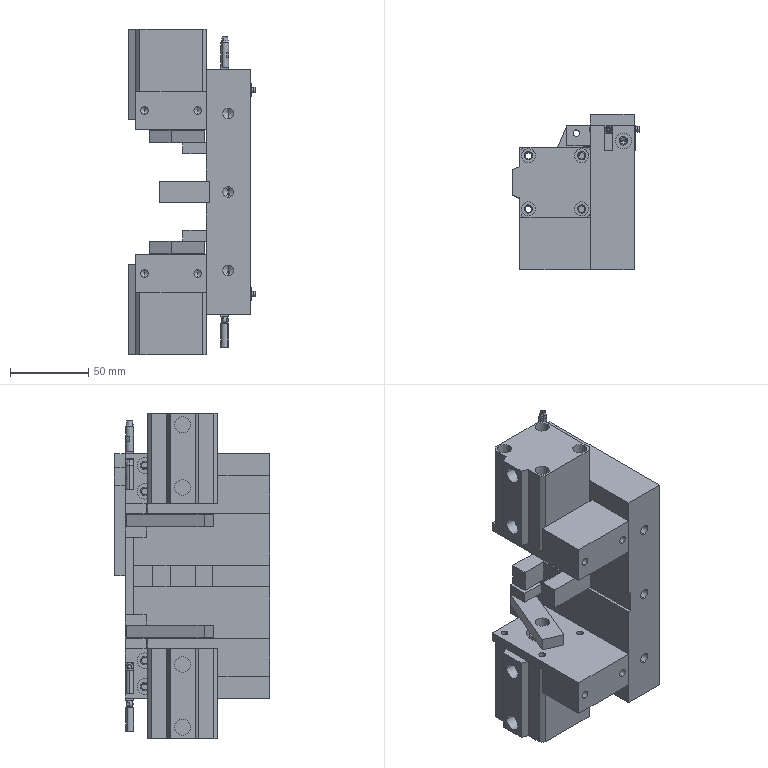Assembly | SolidWorks | mm | 25 component files | 25 solids | 563 faces | box 80.7 x 99 x 208 mm | volume 743615 mm3 | plane 256 | cylinder 242 | cone 53 | sphere 12 | commonest cylinder face diameters 4.2 x44 9 x36 3.5 x24 10 x24 5.5 x20 5.2 x16 4.9 x12 5 x8
Bill of materials:
ACQS-32X25CylinderBody | 2 |  | Square prismatic block with chamfered vertical corners, four corner holes, a larger central bore on the top face, and a trapezoidal tab sticking out from one side.
ACQS-32X25PistonRod | 2 |  | Plain cylindrical tube or sleeve with a concentric bore and flat ends.
InspectionPart | 2 |  | Solid cylindrical pin with a narrow ring-shaped groove of smaller diameter near one end, leaving a short collar at the tip.
PointedHead | 3 |  | Cylindrical shaft with a tapered (conical) end containing a hexagonal socket, a small central hole, and a local flat or recessed step on the side.
PointedHeadBaseA | 1 |  | Rectangular block with an open slot from the top edge, rectangular corner notches, and several holes of different sizes on the large face and on one narrow face.
PointedHeadBaseInsert | 2 |  | Rectangular bar with two round through-holes in a line across the thickness.
PointedHeadDispensingCoverPlateA | 1 |  | Flat rectangular plate with a rectangular notch cut in from one long edge near one end, and two round through-holes along the opposite edge.
PointedHeadDispensingCylinderConnector | 2 |  | Flat bar with two round through-holes of different sizes and one end corner cut at an angle; the outline in plan view is angled or skewed.
PointedHeadDispensingCylinderSeat | 2 |  | Stepped block with an L-shaped side profile: a tall solid section at one end and a thinner plate section with a large bore and four smaller holes.
PointedHeadDispensingMovingPart | 1 |  | Bracket-like solid with two parallel slab sections (lugs) separated by a gap, each with a hole on a shared line, joined to a side wall from which a tall narrow rectangular post rises upward.
PointedHeadDispensingMovingPart1 | 1 |  | Bracket-like solid with two parallel slabs (lugs) separated by a gap, each with a hole on a shared line, joined to a side wall from which a long narrow rectangular post extends downward.
PointedHeadDispensingStopPoint | 1 |  | Rectangular U-shaped block with a rectangular slot running through its full height from one side, plus two holes on one long side face.
PointedHeadInspectionPart | 2 |  | Rectangular block with sharp edges. It has two round holes on perpendicular axes: one runs through from the top face and sits off-center, and the other runs through one side face near one end.
RoundHead | 3 |  | Plain cylindrical shaft. A shoulder steps down to a shorter, narrower neck, which ends in a round ball head. The ball has a round cross-hole whose axis is roughly perpendicular to the shaft axis. The ball outline looks cut by straight edges where the hole opens.
Mates:
1. coincident | PointedHeadDispensingStopPoint-1 face at (12.917, 64.872, -124.387) dir (1, 0, 0) | PointedHeadBaseA-1 face at (12.917, 77.172, -124.387) dir (-1, 0, 0)
2. concentric | PointedHeadDispensingStopPoint-1 face at (12.917, 59.872, -117.387) dir (1, 0, 0) r 2.1 | PointedHeadBaseA-1 face at (38.917, 59.872, -117.387) dir (1, 0, 0) r 2.75
3. concentric | PointedHeadDispensingStopPoint-1 face at (12.917, 31.872, -117.387) dir (1, 0, 0) r 2.1 | PointedHeadBaseA-1 face at (38.917, 31.872, -117.387) dir (1, 0, 0) r 2.75
4. coincident | PointedHeadDispensingMovingPart1-1 face at (25.117, 82.372, -163.887) dir (1, 0, 0) | PointedHeadBaseA-1 face at (25.117, 77.172, -195.387) dir (-1, 0, 0)
5. coincident | PointedHeadDispensingMovingPart1-1 face at (10.917, 77.172, -141.887) dir (0, -1, 0) | PointedHeadBaseA-1 face at (19.917, 77.172, -195.387) dir (0, 1, 0)
6. coincident | PointedHeadDispensingMovingPart-1 face at (25.117, 82.372, -92.887) dir (1, 0, 0) | PointedHeadBaseA-1 face at (25.117, 77.172, -195.387) dir (-1, 0, 0)
7. coincident | PointedHeadDispensingMovingPart-1 face at (10.917, 77.172, -70.887) dir (0, -1, 0) | PointedHeadBaseA-1 face at (19.917, 77.172, -195.387) dir (0, 1, 0)
8. coincident | PointedHeadBaseInsert-1 face at (19.917, 66.172, -163.887) dir (0, -1, 0) | PointedHeadBaseA-1 face at (19.917, 66.172, -39.387) dir (0, 1, 0)
9. concentric | PointedHeadBaseInsert-1 face at (19.917, 69.872, -187.887) dir (-1, 0, 0) r 2.1 | PointedHeadBaseA-1 face at (22.917, 69.872, -187.887) dir (-1, 0, 0) r 2.75
10. concentric | PointedHeadBaseInsert-1 face at (19.917, 69.872, -171.387) dir (-1, 0, 0) r 2.1 | PointedHeadBaseA-1 face at (22.917, 69.872, -171.387) dir (-1, 0, 0) r 2.75
11. coincident | PointedHeadBaseInsert-1 face at (19.917, 77.172, -195.387) dir (-1, 0, 0) | PointedHeadBaseA-1 face at (19.917, 77.172, -195.387) dir (1, 0, 0)
12. coincident | PointedHeadBaseInsert-2 face at (25.117, 77.172, -70.887) dir (1, 0, 0) | PointedHeadBaseA-1 face at (25.117, 77.172, -195.387) dir (-1, 0, 0)
13. concentric | PointedHeadBaseInsert-2 face at (19.917, 69.872, -63.387) dir (-1, 0, 0) r 2.1 | PointedHeadBaseA-1 face at (22.917, 69.872, -63.387) dir (-1, 0, 0) r 2.75
14. concentric | PointedHeadBaseInsert-2 face at (19.917, 69.872, -46.887) dir (-1, 0, 0) r 2.1 | PointedHeadBaseA-1 face at (22.917, 69.872, -46.887) dir (-1, 0, 0) r 2.75
15. concentric | PointedHeadInspectionPart-1 face at (25.617, 79.872, -182.387) dir (1, 0, 0) r 1.75 | InspectionPart-2 face at (42.117, 79.872, -182.387) dir (-1, 0, 0) r 1.75
16. distance | PointedHeadInspectionPart-1 face at (25.617, 82.372, -186.387) dir (-1, 0, 0) | InspectionPart-2 face at (25.117, 79.872, -182.387) dir (-1, 0, 0)
17. coincident | PointedHeadInspectionPart-1 face at (25.617, 82.372, -178.387) dir (0, 0, 1) | PointedHeadBaseA-1 face at (25.117, 50.221, -178.387) dir (0, 0, -1)
18. concentric | PointedHeadInspectionPart-1 face at (32.017, 72.372, -186.387) dir (0, 0, 1) r 2.75 | PointedHeadBaseA-1 face at (32.017, 72.372, -178.387) dir (0, 0, -1) r 2.1
19. concentric | PointedHeadInspectionPart-2 face at (25.617, 79.872, -52.387) dir (1, 0, 0) r 1.75 | InspectionPart-1 face at (42.117, 79.872, -52.387) dir (-1, 0, 0) r 1.75
20. distance | PointedHeadInspectionPart-2 face at (25.617, 82.372, -56.387) dir (-1, 0, 0) | InspectionPart-1 face at (25.117, 79.872, -52.387) dir (-1, 0, 0)
21. coincident | PointedHeadInspectionPart-2 face at (25.617, 82.372, -48.387) dir (0, 0, 1) | PointedHeadBaseA-1 face at (25.117, 50.221, -48.387) dir (0, 0, -1)
22. concentric | PointedHeadInspectionPart-2 face at (32.017, 72.372, -56.387) dir (0, 0, 1) r 2.75 | PointedHeadBaseA-1 face at (32.017, 72.372, -52.587) dir (0, 0, 1) r 5
23. tangent | PointedHead-2 face at (22.667, 79.622, -37.887) dir (0, 0, 1) r 2.45 | InspectionPart-1 face at (25.117, 79.872, -52.387) dir (-1, 0, 0)
24. tangent | PointedHeadBaseInsert-2 face at (19.917, 77.172, -39.387) dir (0, 1, 0) | PointedHead-2 face at (22.667, 79.622, -37.887) dir (0, 0, 1) r 2.45
25. coincident | PointedHeadDispensingMovingPart-1 face at (25.117, 77.172, -37.887) dir (0, 0, 1) | PointedHead-2 face at (22.667, 79.622, -37.887) dir (0, 0, -1)
26. tangent | PointedHead-1 face at (17.767, 79.622, -62.387) dir (0, 0, 1) r 2.45 | PointedHead-3 face at (12.867, 79.622, -62.387) dir (0, 0, 1) r 2.45
27. coincident | PointedHead-1 face at (17.767, 79.622, -62.387) dir (0, 0, -1) | PointedHead-3 face at (12.867, 79.622, -62.387) dir (0, 0, -1)
28. coincident | PointedHeadBaseA-1 face at (19.917, 55.241, -62.387) dir (0, 0, 1) | PointedHead-1 face at (17.767, 79.622, -62.387) dir (0, 0, -1)
29. tangent | PointedHeadBaseA-1 face at (19.917, 77.172, -195.387) dir (0, 1, 0) | PointedHead-3 face at (12.867, 79.622, -62.387) dir (0, 0, 1) r 2.45
30. tangent | PointedHead-1 face at (17.767, 79.622, -62.387) dir (0, 0, 1) r 2.45 | PointedHead-2 face at (22.667, 79.622, -37.887) dir (0, 0, 1) r 2.45
31. tangent | PointedHeadBaseA-1 face at (19.917, 77.172, -195.387) dir (0, 1, 0) | PointedHead-1 face at (17.767, 79.622, -62.387) dir (0, 0, 1) r 2.45
32. tangent | RoundHead-2 face at (17.767, 79.622, -177.387) dir (0, 0, -1) r 2.45 | RoundHead-3 face at (12.867, 79.622, -177.387) dir (0, 0, -1) r 2.45
33. coincident | RoundHead-2 face at (17.767, 79.622, -192.387) dir (0, 0, -1) | RoundHead-3 face at (12.867, 79.622, -192.387) dir (0, 0, -1)
34. tangent | PointedHeadBaseA-1 face at (19.917, 77.172, -195.387) dir (0, 1, 0) | RoundHead-2 face at (17.767, 79.622, -177.387) dir (0, 0, -1) r 2.45
35. tangent | PointedHeadBaseA-1 face at (19.917, 77.172, -195.387) dir (0, 1, 0) | RoundHead-3 face at (12.867, 79.622, -177.387) dir (0, 0, -1) r 2.45
36. tangent | PointedHeadBaseInsert-1 face at (19.917, 77.172, -163.887) dir (0, 1, 0) | RoundHead-1 face at (22.667, 79.622, -201.387) dir (0, 0, -1) r 2.45
37. tangent | RoundHead-1 face at (22.667, 79.622, -201.387) dir (0, 0, -1) r 2.45 | RoundHead-2 face at (17.767, 79.622, -177.387) dir (0, 0, -1) r 2.45
38. tangent | PointedHeadDispensingMovingPart1-1 face at (25.117, 77.172, -196.887) dir (0, 0, -1) | RoundHead-1 face at (22.667, 79.622, -199.137) dir (1, 0, 0) r 2.25
39. coincident | PointedHeadBaseA-1 face at (19.917, 55.241, -192.387) dir (0, 0, 1) | RoundHead-2 face at (17.767, 79.622, -192.387) dir (0, 0, -1)
40. tangent | PointedHeadBaseA-1 face at (25.117, 77.172, -195.387) dir (-1, 0, 0) | RoundHead-1 face at (22.667, 79.622, -201.387) dir (0, 0, -1) r 2.45
41. concentric | PointedHeadDispensingCoverPlateA-1 face at (32.017, 89.372, -102.387) dir (0, 1, 0) r 2.75 | PointedHeadBaseA-1 face at (32.017, 82.372, -102.387) dir (0, 1, 0) r 2.1
42. concentric | PointedHeadDispensingCoverPlateA-1 face at (32.017, 89.372, -72.387) dir (0, 1, 0) r 2.75 | PointedHeadBaseA-1 face at (32.017, 82.372, -72.387) dir (0, 1, 0) r 2.1
43. coincident | PointedHeadDispensingCoverPlateA-1 face at (10.917, 82.372, -39.387) dir (0, -1, 0) | PointedHeadBaseA-1 face at (10.917, 82.372, -39.387) dir (0, 1, 0)
44. parallel | PointedHeadInspectionPart-2 face at (25.617, 82.372, -48.387) dir (0, 1, 0) | PointedHeadDispensingCoverPlateA-1 face at (10.917, 89.372, -39.387) dir (0, 1, 0)
45. width | PointedHeadDispensingCylinderConnector-1 face at (-21.513, 41.37, -156.887) dir (0, 0, -1) | PointedHeadDispensingCylinderConnector-1 face at (-21.513, 41.37, -148.887) dir (0, 0, 1) | PointedHeadDispensingMovingPart1-1 face at (-4.083, 82.372, -156.987) dir (0, 0, 1) | PointedHeadDispensingMovingPart1-1 face at (-4.083, 82.372, -148.787) dir (0, 0, -1)
46. concentric | PointedHeadDispensingCylinderConnector-1 face at (1.917, 77.372, -148.887) dir (0, 0, -1) r 2.1 | PointedHeadDispensingMovingPart1-1 face at (1.917, 77.372, -108.887) dir (0, 0, -1) r 2
47. concentric | PointedHeadDispensingMovingPart-1 face at (1.917, 77.372, -37.887) dir (0, 0, -1) r 2 | PointedHeadDispensingCylinderConnector-2 face at (1.917, 77.372, -77.887) dir (0, 0, -1) r 2.1
48. width | PointedHeadDispensingCylinderConnector-2 face at (-21.513, 41.37, -85.887) dir (0, 0, -1) | PointedHeadDispensingCylinderConnector-2 face at (-21.513, 41.37, -77.887) dir (0, 0, 1) | PointedHeadDispensingMovingPart-1 face at (-4.083, 82.372, -85.987) dir (0, 0, 1) | PointedHeadDispensingMovingPart-1 face at (-4.083, 82.372, -77.787) dir (0, 0, -1)
49. concentric | ACQS-32X25CylinderBody-1 face at (-11.583, 45.872, -198.887) dir (0, 0, 1) r 8 | ACQS-32X25PistonRod-1 face at (-11.583, 45.872, -156.887) dir (0, 0, -1) r 8
50. coincident | PointedHeadDispensingCylinderSeat-2 face at (10.917, 23.372, -163.387) dir (0, 0, -1) | ACQS-32X25CylinderBody-1 face at (10.917, 23.372, -163.387) dir (0, 0, 1)
51. concentric | PointedHeadDispensingCylinderSeat-2 face at (-28.583, 62.872, -163.387) dir (0, 0, -1) r 2.1 | ACQS-32X25CylinderBody-1 face at (-28.583, 62.872, -221.387) dir (0, 0, 1) r 2.6
52. concentric | PointedHeadDispensingCylinderSeat-2 face at (5.417, 62.872, -163.387) dir (0, 0, -1) r 2.1 | ACQS-32X25CylinderBody-1 face at (5.417, 62.872, -221.387) dir (0, 0, 1) r 2.6
53. concentric | ACQS-32X25CylinderBody-2 face at (-11.583, 45.872, -35.887) dir (0, 0, -1) r 8 | ACQS-32X25PistonRod-2 face at (-11.583, 45.872, -77.887) dir (0, 0, 1) r 8
54. coincident | PointedHeadDispensingCylinderSeat-1 face at (-34.083, 23.372, -71.387) dir (0, 0, 1) | ACQS-32X25CylinderBody-2 face at (10.917, 68.372, -71.387) dir (0, 0, -1)
55. concentric | PointedHeadDispensingCylinderSeat-1 face at (-28.583, 62.872, -71.387) dir (0, 0, 1) r 2.1 | ACQS-32X25CylinderBody-2 face at (-28.583, 62.872, -13.387) dir (0, 0, -1) r 2.6
56. concentric | PointedHeadDispensingCylinderSeat-1 face at (5.417, 62.872, -71.387) dir (0, 0, 1) r 2.1 | ACQS-32X25CylinderBody-2 face at (5.417, 62.872, -13.387) dir (0, 0, -1) r 2.6
57. concentric | PointedHeadDispensingCylinderSeat-1 face at (5.417, 28.872, -71.387) dir (0, 0, 1) r 2.1 | ACQS-32X25CylinderBody-2 face at (5.417, 28.872, -13.387) dir (0, 0, -1) r 2.6
58. coincident | PointedHeadBaseA-1 face at (10.917, 82.372, -195.387) dir (-1, 0, 0) | PointedHeadDispensingCylinderSeat-2 face at (10.917, 23.372, -157.387) dir (1, 0, 0)
59. coincident | PointedHeadDispensingCylinderSeat-2 face at (10.917, -9.628, -181.387) dir (0, -1, 0) | PointedHeadBaseA-1 face at (10.917, -9.628, -39.387) dir (0, -1, 0)
60. distance | PointedHeadDispensingCylinderSeat-2 face at (10.917, 23.372, -181.387) dir (0, 0, -1) | PointedHeadBaseA-1 face at (10.917, 82.372, -195.387) dir (0, 0, -1)
61. coincident | PointedHeadDispensingCylinderSeat-1 face at (10.917, 23.372, -77.387) dir (1, 0, 0) | PointedHeadBaseA-1 face at (10.917, 82.372, -195.387) dir (-1, 0, 0)
62. coincident | PointedHeadDispensingCylinderSeat-1 face at (-34.083, -9.628, -53.387) dir (0, -1, 0) | PointedHeadBaseA-1 face at (10.917, -9.628, -39.387) dir (0, -1, 0)
63. distance | PointedHeadDispensingCylinderSeat-1 face at (-34.083, 23.372, -53.387) dir (0, 0, 1) | PointedHeadBaseA-1 face at (10.917, 82.372, -39.387) dir (0, 0, 1)
64. parallel | PointedHeadDispensingCylinderConnector-1 face at (-4.321, 81.872, -148.887) dir (0, 1, 0) | PointedHeadDispensingMovingPart1-1 face at (10.917, 82.372, -141.887) dir (0, 1, 0)
65. coincident | PointedHeadDispensingCylinderConnector-1 face at (-21.513, 41.37, -156.887) dir (0, 0, -1) | ACQS-32X25PistonRod-1 face at (-11.583, 45.872, -156.887) dir (0, 0, 1)
66. parallel | PointedHeadDispensingMovingPart-1 face at (10.917, 82.372, -70.887) dir (0, 1, 0) | PointedHeadDispensingCylinderConnector-2 face at (-4.321, 81.872, -77.887) dir (0, 1, 0)
67. coincident | ACQS-32X25PistonRod-2 face at (-11.583, 45.872, -77.887) dir (0, 0, -1) | PointedHeadDispensingCylinderConnector-2 face at (-21.513, 41.37, -77.887) dir (0, 0, 1)
68. distance | PointedHeadDispensingMovingPart-1 face at (10.917, 82.372, -70.887) dir (0, 0, 1) | PointedHeadBaseA-1 face at (10.917, -16.262, -70.887) dir (0, 0, -1)
69. distance | PointedHeadDispensingMovingPart1-1 face at (10.917, 82.372, -163.887) dir (0, 0, -1) | PointedHeadBaseA-1 face at (10.917, -16.262, -163.887) dir (0, 0, 1)